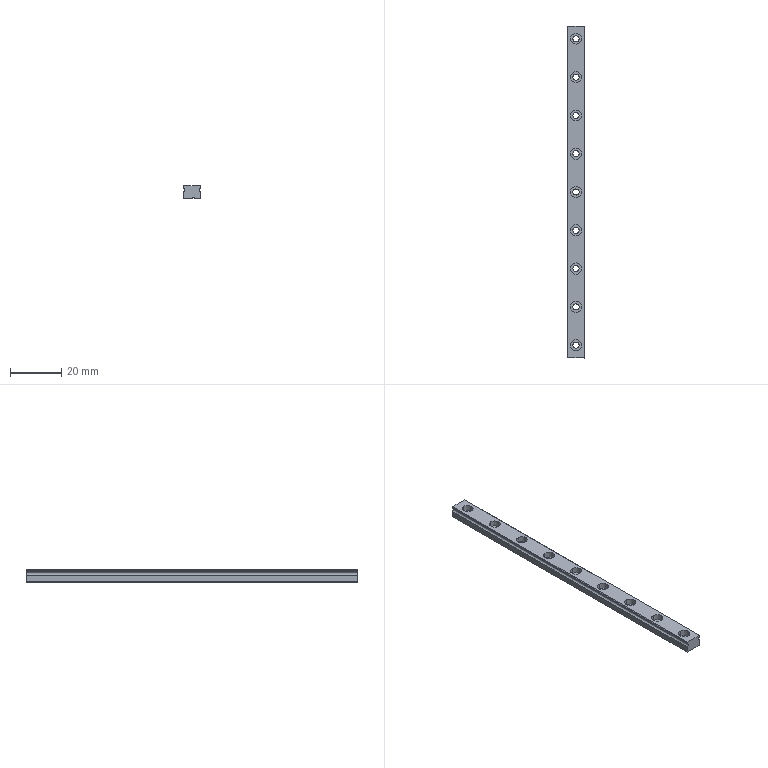Component | SolidWorks | MANIFOLD_SOLID_BREP_40_1-1 | 1 solid | 71 faces | volume 3726 mm3 | cylinder 49 | plane 22 | commonest cylinder face diameters 2.4 x18 4.4 x12 0.6 x10 4.2 x6 1.4 x3